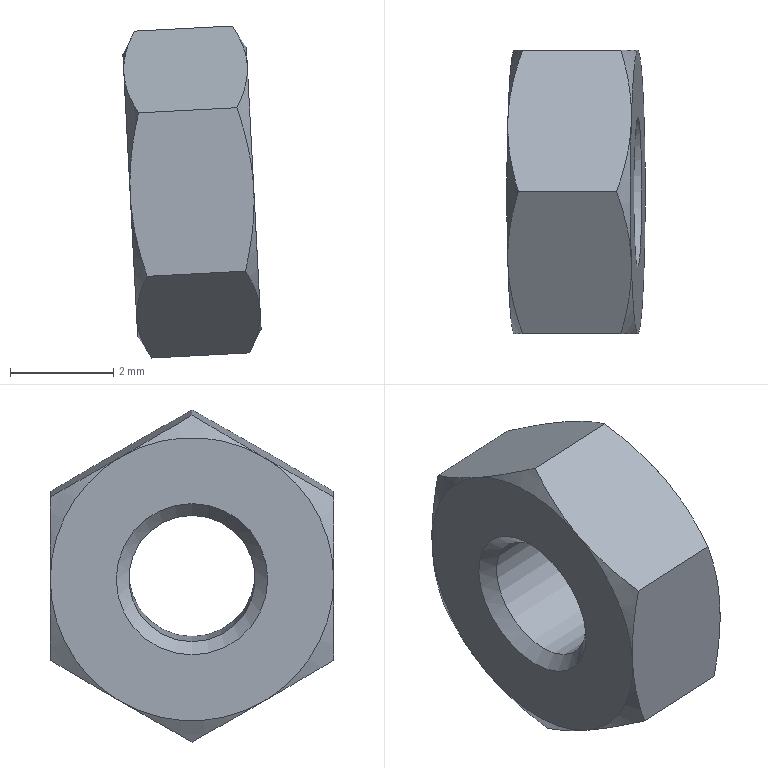Component | NX | GB-T6170_F-2000_M3X0_5 | 1 solid | 23 faces | volume 51 mm3 | cone 14 | plane 8 | cylinder 1 | commonest cylinder face diameters 2.452 x1